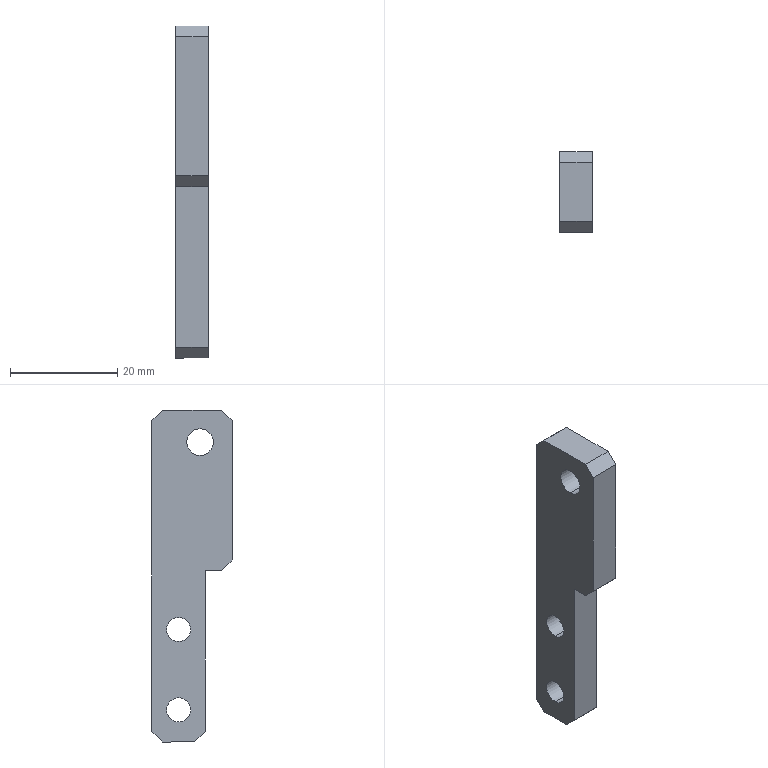Component | SolidWorks | 312981193FloatingJointConnection-1 | 1 solid | 19 faces | box 6 x 15 x 62 mm | volume 4251 mm3 | plane 13 | cylinder 6 | commonest cylinder face diameters 4.5 x4 5 x2 | material Q235-A
build123d program:
from build123d import *

# Parameters (mm, degrees)
BOSS_EXTRUDE1_DEPTH  = 6
M5_TAPPED_HOLE1_D    = 5
CHAMFER1_SIZE        = 2
M4_CLEARANCE_HOLE1_D = 4.5


with BuildPart() as part:
    # Sketch2 → Boss-Extrude1 (new body)
    with BuildSketch(Plane.XY):
        Polygon((-30, 15), (0, 15), (0, 0), (-62, 0), (-62, 10), (-30, 10), align=None)
    extrude(amount=BOSS_EXTRUDE1_DEPTH)

    # M5 Tapped Hole1 (through all)
    with Locations(Plane.XY.offset(6)):
        with Locations((-6, 9)):
            Hole(M5_TAPPED_HOLE1_D / 2)

    # Chamfer1
    chamfer1_edges = [part.edges().sort_by_distance(p)[0] for p in [
        (-30, 15, 3),
        (0, 15, 3),
        (0, 0, 3),
        (-62, 0, 3),
        (-62, 10, 3),
    ]]
    chamfer(chamfer1_edges, length=CHAMFER1_SIZE)

    # M4 Clearance Hole1 (through all)
    with Locations(Plane.XY.offset(6)):
        with Locations((-56, 5), (-41, 5)):
            Hole(M4_CLEARANCE_HOLE1_D / 2)


solid = part.part

# Placed as in the assembly
solid = solid.moved(Location((143.77, 31.768, 86.829), (180, 90, 0)))
STEP:
#1=CARTESIAN_POINT('',(5.66,1.054,1.125));
#2=VERTEX_POINT('',#1);
#3=CARTESIAN_POINT('',(5.66,1.054,1.302));
#4=VERTEX_POINT('',#3);
#5=CARTESIAN_POINT('',(5.66,1.054,1.214));
#6=DIRECTION('',(1.,0.,0.));
#7=DIRECTION('',(0.,0.,1.));
#8=AXIS2_PLACEMENT_3D('',#5,#6,#7);
#9=CIRCLE('',#8,0.08858);
#10=EDGE_CURVE('',#2,#4,#9,.T.);
#11=ORIENTED_EDGE('',*,*,#10,.F.);
#12=CARTESIAN_POINT('',(5.896,1.054,1.125));
#13=VERTEX_POINT('',#12);
#14=CARTESIAN_POINT('',(5.896,1.054,1.125));
#15=DIRECTION('',(1.,0.,0.));
#16=VECTOR('',#15,39.37);
#17=LINE('',#14,#16);
#18=EDGE_CURVE('',#2,#13,#17,.T.);
#19=ORIENTED_EDGE('',*,*,#18,.T.);
#20=CARTESIAN_POINT('',(5.896,1.054,1.302));
#21=VERTEX_POINT('',#20);
#22=CARTESIAN_POINT('',(5.896,1.054,1.214));
#23=DIRECTION('',(1.,0.,0.));
#24=DIRECTION('',(0.,0.,1.));
#25=AXIS2_PLACEMENT_3D('',#22,#23,#24);
#26=CIRCLE('',#25,0.08858);
#27=EDGE_CURVE('',#13,#21,#26,.T.);
#28=ORIENTED_EDGE('',*,*,#27,.T.);
#29=CARTESIAN_POINT('',(5.896,1.054,1.302));
#30=DIRECTION('',(1.,0.,0.));
#31=VECTOR('',#30,39.37);
#32=LINE('',#29,#31);
#33=EDGE_CURVE('',#4,#21,#32,.T.);
#34=ORIENTED_EDGE('',*,*,#33,.F.);
#35=EDGE_LOOP('',(#11,#19,#28,#34));
#36=FACE_OUTER_BOUND('',#35,.T.);
#37=CARTESIAN_POINT('',(5.896,1.054,1.214));
#38=DIRECTION('',(1.,0.,0.));
#39=DIRECTION('',(0.,0.,1.));
#40=AXIS2_PLACEMENT_3D('',#37,#38,#39);
#41=CYLINDRICAL_SURFACE('',#40,0.08858);
#42=ADVANCED_FACE('',(#36),#41,.F.);
#43=CARTESIAN_POINT('',(5.66,1.054,1.716));
#44=VERTEX_POINT('',#43);
#45=CARTESIAN_POINT('',(5.66,1.054,1.893));
#46=VERTEX_POINT('',#45);
#47=CARTESIAN_POINT('',(5.66,1.054,1.804));
#48=DIRECTION('',(1.,0.,0.));
#49=DIRECTION('',(0.,0.,1.));
#50=AXIS2_PLACEMENT_3D('',#47,#48,#49);
#51=CIRCLE('',#50,0.08858);
#52=EDGE_CURVE('',#44,#46,#51,.T.);
#53=ORIENTED_EDGE('',*,*,#52,.F.);
#54=CARTESIAN_POINT('',(5.896,1.054,1.716));
#55=VERTEX_POINT('',#54);
#56=CARTESIAN_POINT('',(5.896,1.054,1.716));
#57=DIRECTION('',(1.,0.,0.));
#58=VECTOR('',#57,39.37);
#59=LINE('',#56,#58);
#60=EDGE_CURVE('',#44,#55,#59,.T.);
#61=ORIENTED_EDGE('',*,*,#60,.T.);
#62=CARTESIAN_POINT('',(5.896,1.054,1.893));
#63=VERTEX_POINT('',#62);
#64=CARTESIAN_POINT('',(5.896,1.054,1.804));
#65=DIRECTION('',(1.,0.,0.));
#66=DIRECTION('',(0.,0.,1.));
#67=AXIS2_PLACEMENT_3D('',#64,#65,#66);
#68=CIRCLE('',#67,0.08858);
#69=EDGE_CURVE('',#55,#63,#68,.T.);
#70=ORIENTED_EDGE('',*,*,#69,.T.);
#71=CARTESIAN_POINT('',(5.896,1.054,1.893));
#72=DIRECTION('',(1.,0.,0.));
#73=VECTOR('',#72,39.37);
#74=LINE('',#71,#73);
#75=EDGE_CURVE('',#46,#63,#74,.T.);
#76=ORIENTED_EDGE('',*,*,#75,.F.);
#77=EDGE_LOOP('',(#53,#61,#70,#76));
#78=FACE_OUTER_BOUND('',#77,.T.);
#79=CARTESIAN_POINT('',(5.896,1.054,1.804));
#80=DIRECTION('',(1.,0.,0.));
#81=DIRECTION('',(0.,0.,1.));
#82=AXIS2_PLACEMENT_3D('',#79,#80,#81);
#83=CYLINDRICAL_SURFACE('',#82,0.08858);
#84=ADVANCED_FACE('',(#78),#83,.F.);
#85=CARTESIAN_POINT('',(5.66,0.8964,3.084));
#86=VERTEX_POINT('',#85);
#87=CARTESIAN_POINT('',(5.66,0.8964,3.281));
#88=VERTEX_POINT('',#87);
#89=CARTESIAN_POINT('',(5.66,0.8964,3.182));
#90=DIRECTION('',(1.,0.,0.));
#91=DIRECTION('',(0.,0.,1.));
#92=AXIS2_PLACEMENT_3D('',#89,#90,#91);
#93=CIRCLE('',#92,0.09843);
#94=EDGE_CURVE('',#86,#88,#93,.T.);
#95=ORIENTED_EDGE('',*,*,#94,.F.);
#96=CARTESIAN_POINT('',(5.896,0.8964,3.084));
#97=VERTEX_POINT('',#96);
#98=CARTESIAN_POINT('',(5.896,0.8964,3.084));
#99=DIRECTION('',(1.,0.,0.));
#100=VECTOR('',#99,39.37);
#101=LINE('',#98,#100);
#102=EDGE_CURVE('',#86,#97,#101,.T.);
#103=ORIENTED_EDGE('',*,*,#102,.T.);
#104=CARTESIAN_POINT('',(5.896,0.8964,3.281));
#105=VERTEX_POINT('',#104);
#106=CARTESIAN_POINT('',(5.896,0.8964,3.182));
#107=DIRECTION('',(1.,0.,0.));
#108=DIRECTION('',(0.,0.,1.));
#109=AXIS2_PLACEMENT_3D('',#106,#107,#108);
#110=CIRCLE('',#109,0.09843);
#111=EDGE_CURVE('',#97,#105,#110,.T.);
#112=ORIENTED_EDGE('',*,*,#111,.T.);
#113=CARTESIAN_POINT('',(5.896,0.8964,3.281));
#114=DIRECTION('',(1.,0.,0.));
#115=VECTOR('',#114,39.37);
#116=LINE('',#113,#115);
#117=EDGE_CURVE('',#88,#105,#116,.T.);
#118=ORIENTED_EDGE('',*,*,#117,.F.);
#119=EDGE_LOOP('',(#95,#103,#112,#118));
#120=FACE_OUTER_BOUND('',#119,.T.);
#121=CARTESIAN_POINT('',(5.896,0.8964,3.182));
#122=DIRECTION('',(1.,0.,0.));
#123=DIRECTION('',(0.,0.,1.));
#124=AXIS2_PLACEMENT_3D('',#121,#122,#123);
#125=CYLINDRICAL_SURFACE('',#124,0.09843);
#126=ADVANCED_FACE('',(#120),#125,.F.);
#127=CARTESIAN_POINT('',(5.896,0.7389,2.237));
#128=VERTEX_POINT('',#127);
#129=CARTESIAN_POINT('',(5.896,0.857,2.237));
#130=VERTEX_POINT('',#129);
#131=CARTESIAN_POINT('',(5.896,0.6602,2.237));
#132=DIRECTION('',(-0.,1.,-0.));
#133=VECTOR('',#132,39.37);
#134=LINE('',#131,#133);
#135=EDGE_CURVE('',#128,#130,#134,.T.);
#136=ORIENTED_EDGE('',*,*,#135,.F.);
#137=CARTESIAN_POINT('',(5.66,0.7389,2.237));
#138=VERTEX_POINT('',#137);
#139=CARTESIAN_POINT('',(5.896,0.7389,2.237));
#140=DIRECTION('',(-1.,-0.,-0.));
#141=VECTOR('',#140,39.37);
#142=LINE('',#139,#141);
#143=EDGE_CURVE('',#128,#138,#142,.T.);
#144=ORIENTED_EDGE('',*,*,#143,.T.);
#145=CARTESIAN_POINT('',(5.66,0.857,2.237));
#146=VERTEX_POINT('',#145);
#147=CARTESIAN_POINT('',(5.66,0.6602,2.237));
#148=DIRECTION('',(-0.,1.,-0.));
#149=VECTOR('',#148,39.37);
#150=LINE('',#147,#149);
#151=EDGE_CURVE('',#138,#146,#150,.T.);
#152=ORIENTED_EDGE('',*,*,#151,.T.);
#153=CARTESIAN_POINT('',(5.896,0.857,2.237));
#154=DIRECTION('',(-1.,-0.,-0.));
#155=VECTOR('',#154,39.37);
#156=LINE('',#153,#155);
#157=EDGE_CURVE('',#130,#146,#156,.T.);
#158=ORIENTED_EDGE('',*,*,#157,.F.);
#159=EDGE_LOOP('',(#136,#144,#152,#158));
#160=FACE_OUTER_BOUND('',#159,.T.);
#161=CARTESIAN_POINT('',(5.896,0.6602,2.237));
#162=DIRECTION('',(-0.,0.,1.));
#163=DIRECTION('',(-1.,-0.,-0.));
#164=AXIS2_PLACEMENT_3D('',#161,#162,#163);
#165=PLANE('',#164);
#166=ADVANCED_FACE('',(#160),#165,.F.);
#167=CARTESIAN_POINT('',(5.66,0.857,1.056));
#168=VERTEX_POINT('',#167);
#169=CARTESIAN_POINT('',(5.66,0.857,0.9775));
#170=DIRECTION('',(0.,-0.,-1.));
#171=VECTOR('',#170,39.37);
#172=LINE('',#169,#171);
#173=EDGE_CURVE('',#146,#168,#172,.T.);
#174=ORIENTED_EDGE('',*,*,#173,.T.);
#175=CARTESIAN_POINT('',(5.896,0.857,1.056));
#176=VERTEX_POINT('',#175);
#177=CARTESIAN_POINT('',(5.896,0.857,1.056));
#178=DIRECTION('',(1.,0.,0.));
#179=VECTOR('',#178,39.37);
#180=LINE('',#177,#179);
#181=EDGE_CURVE('',#168,#176,#180,.T.);
#182=ORIENTED_EDGE('',*,*,#181,.T.);
#183=CARTESIAN_POINT('',(5.896,0.857,0.9775));
#184=DIRECTION('',(0.,-0.,-1.));
#185=VECTOR('',#184,39.37);
#186=LINE('',#183,#185);
#187=EDGE_CURVE('',#130,#176,#186,.T.);
#188=ORIENTED_EDGE('',*,*,#187,.F.);
#189=ORIENTED_EDGE('',*,*,#157,.T.);
#190=EDGE_LOOP('',(#174,#182,#188,#189));
#191=FACE_OUTER_BOUND('',#190,.T.);
#192=CARTESIAN_POINT('',(5.896,0.857,0.9775));
#193=DIRECTION('',(-0.,1.,-0.));
#194=DIRECTION('',(-1.,-0.,-0.));
#195=AXIS2_PLACEMENT_3D('',#192,#193,#194);
#196=PLANE('',#195);
#197=ADVANCED_FACE('',(#191),#196,.F.);
#198=CARTESIAN_POINT('',(5.66,0.9358,0.9775));
#199=VERTEX_POINT('',#198);
#200=CARTESIAN_POINT('',(5.66,1.172,0.9775));
#201=VERTEX_POINT('',#200);
#202=CARTESIAN_POINT('',(5.66,1.251,0.9775));
#203=DIRECTION('',(-0.,1.,-0.));
#204=VECTOR('',#203,39.37);
#205=LINE('',#202,#204);
#206=EDGE_CURVE('',#199,#201,#205,.T.);
#207=ORIENTED_EDGE('',*,*,#206,.T.);
#208=CARTESIAN_POINT('',(5.896,1.172,0.9775));
#209=VERTEX_POINT('',#208);
#210=CARTESIAN_POINT('',(5.896,1.172,0.9775));
#211=DIRECTION('',(1.,0.,0.));
#212=VECTOR('',#211,39.37);
#213=LINE('',#210,#212);
#214=EDGE_CURVE('',#201,#209,#213,.T.);
#215=ORIENTED_EDGE('',*,*,#214,.T.);
#216=CARTESIAN_POINT('',(5.896,0.9358,0.9775));
#217=VERTEX_POINT('',#216);
#218=CARTESIAN_POINT('',(5.896,1.251,0.9775));
#219=DIRECTION('',(-0.,1.,-0.));
#220=VECTOR('',#219,39.37);
#221=LINE('',#218,#220);
#222=EDGE_CURVE('',#217,#209,#221,.T.);
#223=ORIENTED_EDGE('',*,*,#222,.F.);
#224=CARTESIAN_POINT('',(5.896,0.9358,0.9775));
#225=DIRECTION('',(-1.,-0.,-0.));
#226=VECTOR('',#225,39.37);
#227=LINE('',#224,#226);
#228=EDGE_CURVE('',#217,#199,#227,.T.);
#229=ORIENTED_EDGE('',*,*,#228,.T.);
#230=EDGE_LOOP('',(#207,#215,#223,#229));
#231=FACE_OUTER_BOUND('',#230,.T.);
#232=CARTESIAN_POINT('',(5.896,1.251,0.9775));
#233=DIRECTION('',(-0.,0.,1.));
#234=DIRECTION('',(-1.,-0.,-0.));
#235=AXIS2_PLACEMENT_3D('',#232,#233,#234);
#236=PLANE('',#235);
#237=ADVANCED_FACE('',(#231),#236,.F.);
#238=CARTESIAN_POINT('',(5.896,1.251,1.056));
#239=VERTEX_POINT('',#238);
#240=CARTESIAN_POINT('',(5.896,1.251,3.34));
#241=VERTEX_POINT('',#240);
#242=CARTESIAN_POINT('',(5.896,1.251,0.9775));
#243=DIRECTION('',(-0.,0.,1.));
#244=VECTOR('',#243,39.37);
#245=LINE('',#242,#244);
#246=EDGE_CURVE('',#239,#241,#245,.T.);
#247=ORIENTED_EDGE('',*,*,#246,.F.);
#248=CARTESIAN_POINT('',(5.66,1.251,1.056));
#249=VERTEX_POINT('',#248);
#250=CARTESIAN_POINT('',(5.896,1.251,1.056));
#251=DIRECTION('',(-1.,-0.,-0.));
#252=VECTOR('',#251,39.37);
#253=LINE('',#250,#252);
#254=EDGE_CURVE('',#239,#249,#253,.T.);
#255=ORIENTED_EDGE('',*,*,#254,.T.);
#256=CARTESIAN_POINT('',(5.66,1.251,3.34));
#257=VERTEX_POINT('',#256);
#258=CARTESIAN_POINT('',(5.66,1.251,0.9775));
#259=DIRECTION('',(-0.,0.,1.));
#260=VECTOR('',#259,39.37);
#261=LINE('',#258,#260);
#262=EDGE_CURVE('',#249,#257,#261,.T.);
#263=ORIENTED_EDGE('',*,*,#262,.T.);
#264=CARTESIAN_POINT('',(5.896,1.251,3.34));
#265=DIRECTION('',(1.,0.,0.));
#266=VECTOR('',#265,39.37);
#267=LINE('',#264,#266);
#268=EDGE_CURVE('',#257,#241,#267,.T.);
#269=ORIENTED_EDGE('',*,*,#268,.T.);
#270=EDGE_LOOP('',(#247,#255,#263,#269));
#271=FACE_OUTER_BOUND('',#270,.T.);
#272=CARTESIAN_POINT('',(5.896,1.251,0.9775));
#273=DIRECTION('',(0.,-1.,0.));
#274=DIRECTION('',(1.,0.,0.));
#275=AXIS2_PLACEMENT_3D('',#272,#273,#274);
#276=PLANE('',#275);
#277=ADVANCED_FACE('',(#271),#276,.F.);
#278=CARTESIAN_POINT('',(5.896,1.172,3.418));
#279=VERTEX_POINT('',#278);
#280=CARTESIAN_POINT('',(5.896,0.7389,3.418));
#281=VERTEX_POINT('',#280);
#282=CARTESIAN_POINT('',(5.896,0.6602,3.418));
#283=DIRECTION('',(0.,-1.,0.));
#284=VECTOR('',#283,39.37);
#285=LINE('',#282,#284);
#286=EDGE_CURVE('',#279,#281,#285,.T.);
#287=ORIENTED_EDGE('',*,*,#286,.F.);
#288=CARTESIAN_POINT('',(5.66,1.172,3.418));
#289=VERTEX_POINT('',#288);
#290=CARTESIAN_POINT('',(5.896,1.172,3.418));
#291=DIRECTION('',(-1.,-0.,-0.));
#292=VECTOR('',#291,39.37);
#293=LINE('',#290,#292);
#294=EDGE_CURVE('',#279,#289,#293,.T.);
#295=ORIENTED_EDGE('',*,*,#294,.T.);
#296=CARTESIAN_POINT('',(5.66,0.7389,3.418));
#297=VERTEX_POINT('',#296);
#298=CARTESIAN_POINT('',(5.66,0.6602,3.418));
#299=DIRECTION('',(0.,-1.,0.));
#300=VECTOR('',#299,39.37);
#301=LINE('',#298,#300);
#302=EDGE_CURVE('',#289,#297,#301,.T.);
#303=ORIENTED_EDGE('',*,*,#302,.T.);
#304=CARTESIAN_POINT('',(5.896,0.7389,3.418));
#305=DIRECTION('',(1.,0.,0.));
#306=VECTOR('',#305,39.37);
#307=LINE('',#304,#306);
#308=EDGE_CURVE('',#297,#281,#307,.T.);
#309=ORIENTED_EDGE('',*,*,#308,.T.);
#310=EDGE_LOOP('',(#287,#295,#303,#309));
#311=FACE_OUTER_BOUND('',#310,.T.);
#312=CARTESIAN_POINT('',(5.896,0.6602,3.418));
#313=DIRECTION('',(0.,-0.,-1.));
#314=DIRECTION('',(-0.,1.,-0.));
#315=AXIS2_PLACEMENT_3D('',#312,#313,#314);
#316=PLANE('',#315);
#317=ADVANCED_FACE('',(#311),#316,.F.);
#318=CARTESIAN_POINT('',(5.66,0.6602,3.34));
#319=VERTEX_POINT('',#318);
#320=CARTESIAN_POINT('',(5.66,0.6602,2.316));
#321=VERTEX_POINT('',#320);
#322=CARTESIAN_POINT('',(5.66,0.6602,2.237));
#323=DIRECTION('',(0.,-0.,-1.));
#324=VECTOR('',#323,39.37);
#325=LINE('',#322,#324);
#326=EDGE_CURVE('',#319,#321,#325,.T.);
#327=ORIENTED_EDGE('',*,*,#326,.T.);
#328=CARTESIAN_POINT('',(5.896,0.6602,2.316));
#329=VERTEX_POINT('',#328);
#330=CARTESIAN_POINT('',(5.896,0.6602,2.316));
#331=DIRECTION('',(1.,0.,0.));
#332=VECTOR('',#331,39.37);
#333=LINE('',#330,#332);
#334=EDGE_CURVE('',#321,#329,#333,.T.);
#335=ORIENTED_EDGE('',*,*,#334,.T.);
#336=CARTESIAN_POINT('',(5.896,0.6602,3.34));
#337=VERTEX_POINT('',#336);
#338=CARTESIAN_POINT('',(5.896,0.6602,2.237));
#339=DIRECTION('',(0.,-0.,-1.));
#340=VECTOR('',#339,39.37);
#341=LINE('',#338,#340);
#342=EDGE_CURVE('',#337,#329,#341,.T.);
#343=ORIENTED_EDGE('',*,*,#342,.F.);
#344=CARTESIAN_POINT('',(5.896,0.6602,3.34));
#345=DIRECTION('',(-1.,-0.,-0.));
#346=VECTOR('',#345,39.37);
#347=LINE('',#344,#346);
#348=EDGE_CURVE('',#337,#319,#347,.T.);
#349=ORIENTED_EDGE('',*,*,#348,.T.);
#350=EDGE_LOOP('',(#327,#335,#343,#349));
#351=FACE_OUTER_BOUND('',#350,.T.);
#352=CARTESIAN_POINT('',(5.896,0.6602,2.237));
#353=DIRECTION('',(-0.,1.,-0.));
#354=DIRECTION('',(-1.,-0.,-0.));
#355=AXIS2_PLACEMENT_3D('',#352,#353,#354);
#356=PLANE('',#355);
#357=ADVANCED_FACE('',(#351),#356,.F.);
#358=CARTESIAN_POINT('',(5.896,1.054,1.214));
#359=DIRECTION('',(1.,0.,0.));
#360=DIRECTION('',(0.,0.,1.));
#361=AXIS2_PLACEMENT_3D('',#358,#359,#360);
#362=CIRCLE('',#361,0.08858);
#363=EDGE_CURVE('',#21,#13,#362,.T.);
#364=ORIENTED_EDGE('',*,*,#363,.F.);
#365=ORIENTED_EDGE('',*,*,#27,.F.);
#366=EDGE_LOOP('',(#364,#365));
#367=FACE_BOUND('',#366,.T.);
#368=CARTESIAN_POINT('',(5.896,1.054,1.804));
#369=DIRECTION('',(1.,0.,0.));
#370=DIRECTION('',(0.,0.,1.));
#371=AXIS2_PLACEMENT_3D('',#368,#369,#370);
#372=CIRCLE('',#371,0.08858);
#373=EDGE_CURVE('',#63,#55,#372,.T.);
#374=ORIENTED_EDGE('',*,*,#373,.F.);
#375=ORIENTED_EDGE('',*,*,#69,.F.);
#376=EDGE_LOOP('',(#374,#375));
#377=FACE_BOUND('',#376,.T.);
#378=CARTESIAN_POINT('',(5.896,0.8964,3.182));
#379=DIRECTION('',(1.,0.,0.));
#380=DIRECTION('',(0.,0.,1.));
#381=AXIS2_PLACEMENT_3D('',#378,#379,#380);
#382=CIRCLE('',#381,0.09843);
#383=EDGE_CURVE('',#105,#97,#382,.T.);
#384=ORIENTED_EDGE('',*,*,#383,.F.);
#385=ORIENTED_EDGE('',*,*,#111,.F.);
#386=EDGE_LOOP('',(#384,#385));
#387=FACE_BOUND('',#386,.T.);
#388=ORIENTED_EDGE('',*,*,#222,.T.);
#389=CARTESIAN_POINT('',(5.896,1.644,1.45));
#390=DIRECTION('',(-0.,0.7071,0.7071));
#391=VECTOR('',#390,39.37);
#392=LINE('',#389,#391);
#393=EDGE_CURVE('',#209,#239,#392,.T.);
#394=ORIENTED_EDGE('',*,*,#393,.T.);
#395=ORIENTED_EDGE('',*,*,#246,.T.);
#396=CARTESIAN_POINT('',(5.896,1.605,2.985));
#397=DIRECTION('',(-0.,-0.7071,0.7071));
#398=VECTOR('',#397,39.37);
#399=LINE('',#396,#398);
#400=EDGE_CURVE('',#241,#279,#399,.T.);
#401=ORIENTED_EDGE('',*,*,#400,.T.);
#402=ORIENTED_EDGE('',*,*,#286,.T.);
#403=CARTESIAN_POINT('',(5.896,0.2074,2.887));
#404=DIRECTION('',(0.,-0.7071,-0.7071));
#405=VECTOR('',#404,39.37);
#406=LINE('',#403,#405);
#407=EDGE_CURVE('',#281,#337,#406,.T.);
#408=ORIENTED_EDGE('',*,*,#407,.T.);
#409=ORIENTED_EDGE('',*,*,#342,.T.);
#410=CARTESIAN_POINT('',(5.896,0.798,2.178));
#411=DIRECTION('',(0.,0.7071,-0.7071));
#412=VECTOR('',#411,39.37);
#413=LINE('',#410,#412);
#414=EDGE_CURVE('',#329,#128,#413,.T.);
#415=ORIENTED_EDGE('',*,*,#414,.T.);
#416=ORIENTED_EDGE('',*,*,#135,.T.);
#417=ORIENTED_EDGE('',*,*,#187,.T.);
#418=CARTESIAN_POINT('',(5.896,0.2665,1.647));
#419=DIRECTION('',(0.,0.7071,-0.7071));
#420=VECTOR('',#419,39.37);
#421=LINE('',#418,#420);
#422=EDGE_CURVE('',#176,#217,#421,.T.);
#423=ORIENTED_EDGE('',*,*,#422,.T.);
#424=EDGE_LOOP('',(#388,#394,#395,#401,#402,#408,#409,#415,#416,#417,#423));
#425=FACE_OUTER_BOUND('',#424,.T.);
#426=CARTESIAN_POINT('',(5.896,0.857,2.237));
#427=DIRECTION('',(1.,0.,0.));
#428=DIRECTION('',(-0.,0.,1.));
#429=AXIS2_PLACEMENT_3D('',#426,#427,#428);
#430=PLANE('',#429);
#431=ADVANCED_FACE('',(#367,#377,#387,#425),#430,.T.);
#432=CARTESIAN_POINT('',(5.66,1.054,1.214));
#433=DIRECTION('',(1.,0.,0.));
#434=DIRECTION('',(0.,0.,1.));
#435=AXIS2_PLACEMENT_3D('',#432,#433,#434);
#436=CIRCLE('',#435,0.08858);
#437=EDGE_CURVE('',#4,#2,#436,.T.);
#438=ORIENTED_EDGE('',*,*,#437,.T.);
#439=ORIENTED_EDGE('',*,*,#10,.T.);
#440=EDGE_LOOP('',(#438,#439));
#441=FACE_BOUND('',#440,.T.);
#442=CARTESIAN_POINT('',(5.66,1.054,1.804));
#443=DIRECTION('',(1.,0.,0.));
#444=DIRECTION('',(0.,0.,1.));
#445=AXIS2_PLACEMENT_3D('',#442,#443,#444);
#446=CIRCLE('',#445,0.08858);
#447=EDGE_CURVE('',#46,#44,#446,.T.);
#448=ORIENTED_EDGE('',*,*,#447,.T.);
#449=ORIENTED_EDGE('',*,*,#52,.T.);
#450=EDGE_LOOP('',(#448,#449));
#451=FACE_BOUND('',#450,.T.);
#452=CARTESIAN_POINT('',(5.66,0.8964,3.182));
#453=DIRECTION('',(1.,0.,0.));
#454=DIRECTION('',(0.,0.,1.));
#455=AXIS2_PLACEMENT_3D('',#452,#453,#454);
#456=CIRCLE('',#455,0.09843);
#457=EDGE_CURVE('',#88,#86,#456,.T.);
#458=ORIENTED_EDGE('',*,*,#457,.T.);
#459=ORIENTED_EDGE('',*,*,#94,.T.);
#460=EDGE_LOOP('',(#458,#459));
#461=FACE_BOUND('',#460,.T.);
#462=ORIENTED_EDGE('',*,*,#262,.F.);
#463=CARTESIAN_POINT('',(5.66,1.251,1.056));
#464=DIRECTION('',(0.,-0.7071,-0.7071));
#465=VECTOR('',#464,39.37);
#466=LINE('',#463,#465);
#467=EDGE_CURVE('',#249,#201,#466,.T.);
#468=ORIENTED_EDGE('',*,*,#467,.T.);
#469=ORIENTED_EDGE('',*,*,#206,.F.);
#470=CARTESIAN_POINT('',(5.66,0.9358,0.9775));
#471=DIRECTION('',(-0.,-0.7071,0.7071));
#472=VECTOR('',#471,39.37);
#473=LINE('',#470,#472);
#474=EDGE_CURVE('',#199,#168,#473,.T.);
#475=ORIENTED_EDGE('',*,*,#474,.T.);
#476=ORIENTED_EDGE('',*,*,#173,.F.);
#477=ORIENTED_EDGE('',*,*,#151,.F.);
#478=CARTESIAN_POINT('',(5.66,0.7389,2.237));
#479=DIRECTION('',(-0.,-0.7071,0.7071));
#480=VECTOR('',#479,39.37);
#481=LINE('',#478,#480);
#482=EDGE_CURVE('',#138,#321,#481,.T.);
#483=ORIENTED_EDGE('',*,*,#482,.T.);
#484=ORIENTED_EDGE('',*,*,#326,.F.);
#485=CARTESIAN_POINT('',(5.66,0.6602,3.34));
#486=DIRECTION('',(-0.,0.7071,0.7071));
#487=VECTOR('',#486,39.37);
#488=LINE('',#485,#487);
#489=EDGE_CURVE('',#319,#297,#488,.T.);
#490=ORIENTED_EDGE('',*,*,#489,.T.);
#491=ORIENTED_EDGE('',*,*,#302,.F.);
#492=CARTESIAN_POINT('',(5.66,1.172,3.418));
#493=DIRECTION('',(0.,0.7071,-0.7071));
#494=VECTOR('',#493,39.37);
#495=LINE('',#492,#494);
#496=EDGE_CURVE('',#289,#257,#495,.T.);
#497=ORIENTED_EDGE('',*,*,#496,.T.);
#498=EDGE_LOOP('',(#462,#468,#469,#475,#476,#477,#483,#484,#490,#491,#497));
#499=FACE_OUTER_BOUND('',#498,.T.);
#500=CARTESIAN_POINT('',(5.66,0.857,2.237));
#501=DIRECTION('',(1.,0.,0.));
#502=DIRECTION('',(-0.,0.,1.));
#503=AXIS2_PLACEMENT_3D('',#500,#501,#502);
#504=PLANE('',#503);
#505=ADVANCED_FACE('',(#441,#451,#461,#499),#504,.F.);
#506=ORIENTED_EDGE('',*,*,#102,.F.);
#507=ORIENTED_EDGE('',*,*,#457,.F.);
#508=ORIENTED_EDGE('',*,*,#117,.T.);
#509=ORIENTED_EDGE('',*,*,#383,.T.);
#510=EDGE_LOOP('',(#506,#507,#508,#509));
#511=FACE_OUTER_BOUND('',#510,.T.);
#512=CARTESIAN_POINT('',(5.896,0.8964,3.182));
#513=DIRECTION('',(1.,0.,0.));
#514=DIRECTION('',(0.,0.,1.));
#515=AXIS2_PLACEMENT_3D('',#512,#513,#514);
#516=CYLINDRICAL_SURFACE('',#515,0.09843);
#517=ADVANCED_FACE('',(#511),#516,.F.);
#518=ORIENTED_EDGE('',*,*,#393,.F.);
#519=ORIENTED_EDGE('',*,*,#214,.F.);
#520=ORIENTED_EDGE('',*,*,#467,.F.);
#521=ORIENTED_EDGE('',*,*,#254,.F.);
#522=EDGE_LOOP('',(#518,#519,#520,#521));
#523=FACE_OUTER_BOUND('',#522,.T.);
#524=CARTESIAN_POINT('',(5.896,1.251,1.056));
#525=DIRECTION('',(-0.,-0.7071,0.7071));
#526=DIRECTION('',(0.,-0.7071,-0.7071));
#527=AXIS2_PLACEMENT_3D('',#524,#525,#526);
#528=PLANE('',#527);
#529=ADVANCED_FACE('',(#523),#528,.F.);
#530=ORIENTED_EDGE('',*,*,#422,.F.);
#531=ORIENTED_EDGE('',*,*,#181,.F.);
#532=ORIENTED_EDGE('',*,*,#474,.F.);
#533=ORIENTED_EDGE('',*,*,#228,.F.);
#534=EDGE_LOOP('',(#530,#531,#532,#533));
#535=FACE_OUTER_BOUND('',#534,.T.);
#536=CARTESIAN_POINT('',(5.896,0.9358,0.9775));
#537=DIRECTION('',(-0.,0.7071,0.7071));
#538=DIRECTION('',(-0.,-0.7071,0.7071));
#539=AXIS2_PLACEMENT_3D('',#536,#537,#538);
#540=PLANE('',#539);
#541=ADVANCED_FACE('',(#535),#540,.F.);
#542=ORIENTED_EDGE('',*,*,#414,.F.);
#543=ORIENTED_EDGE('',*,*,#334,.F.);
#544=ORIENTED_EDGE('',*,*,#482,.F.);
#545=ORIENTED_EDGE('',*,*,#143,.F.);
#546=EDGE_LOOP('',(#542,#543,#544,#545));
#547=FACE_OUTER_BOUND('',#546,.T.);
#548=CARTESIAN_POINT('',(5.896,0.7389,2.237));
#549=DIRECTION('',(-0.,0.7071,0.7071));
#550=DIRECTION('',(-0.,-0.7071,0.7071));
#551=AXIS2_PLACEMENT_3D('',#548,#549,#550);
#552=PLANE('',#551);
#553=ADVANCED_FACE('',(#547),#552,.F.);
#554=ORIENTED_EDGE('',*,*,#400,.F.);
#555=ORIENTED_EDGE('',*,*,#268,.F.);
#556=ORIENTED_EDGE('',*,*,#496,.F.);
#557=ORIENTED_EDGE('',*,*,#294,.F.);
#558=EDGE_LOOP('',(#554,#555,#556,#557));
#559=FACE_OUTER_BOUND('',#558,.T.);
#560=CARTESIAN_POINT('',(5.896,1.172,3.418));
#561=DIRECTION('',(0.,-0.7071,-0.7071));
#562=DIRECTION('',(0.,0.7071,-0.7071));
#563=AXIS2_PLACEMENT_3D('',#560,#561,#562);
#564=PLANE('',#563);
#565=ADVANCED_FACE('',(#559),#564,.F.);
#566=ORIENTED_EDGE('',*,*,#407,.F.);
#567=ORIENTED_EDGE('',*,*,#308,.F.);
#568=ORIENTED_EDGE('',*,*,#489,.F.);
#569=ORIENTED_EDGE('',*,*,#348,.F.);
#570=EDGE_LOOP('',(#566,#567,#568,#569));
#571=FACE_OUTER_BOUND('',#570,.T.);
#572=CARTESIAN_POINT('',(5.896,0.6602,3.34));
#573=DIRECTION('',(0.,0.7071,-0.7071));
#574=DIRECTION('',(-0.,0.7071,0.7071));
#575=AXIS2_PLACEMENT_3D('',#572,#573,#574);
#576=PLANE('',#575);
#577=ADVANCED_FACE('',(#571),#576,.F.);
#578=ORIENTED_EDGE('',*,*,#60,.F.);
#579=ORIENTED_EDGE('',*,*,#447,.F.);
#580=ORIENTED_EDGE('',*,*,#75,.T.);
#581=ORIENTED_EDGE('',*,*,#373,.T.);
#582=EDGE_LOOP('',(#578,#579,#580,#581));
#583=FACE_OUTER_BOUND('',#582,.T.);
#584=CARTESIAN_POINT('',(5.896,1.054,1.804));
#585=DIRECTION('',(1.,0.,0.));
#586=DIRECTION('',(0.,0.,1.));
#587=AXIS2_PLACEMENT_3D('',#584,#585,#586);
#588=CYLINDRICAL_SURFACE('',#587,0.08858);
#589=ADVANCED_FACE('',(#583),#588,.F.);
#590=ORIENTED_EDGE('',*,*,#18,.F.);
#591=ORIENTED_EDGE('',*,*,#437,.F.);
#592=ORIENTED_EDGE('',*,*,#33,.T.);
#593=ORIENTED_EDGE('',*,*,#363,.T.);
#594=EDGE_LOOP('',(#590,#591,#592,#593));
#595=FACE_OUTER_BOUND('',#594,.T.);
#596=CARTESIAN_POINT('',(5.896,1.054,1.214));
#597=DIRECTION('',(1.,0.,0.));
#598=DIRECTION('',(0.,0.,1.));
#599=AXIS2_PLACEMENT_3D('',#596,#597,#598);
#600=CYLINDRICAL_SURFACE('',#599,0.08858);
#601=ADVANCED_FACE('',(#595),#600,.F.);
#602=CLOSED_SHELL('',(#42,#84,#126,#166,#197,#237,#277,#317,#357,#431,#505,#517,#529,#541,#553,#565,#577,#589,#601));
#603=MANIFOLD_SOLID_BREP('',#602);
#604=CARTESIAN_POINT('',(0.,0.,0.));
#605=DIRECTION('',(0.,0.,1.));
#606=DIRECTION('',(1.,0.,0.));
#607=AXIS2_PLACEMENT_3D('',#604,#605,#606);
#608=(LENGTH_UNIT()NAMED_UNIT(*)SI_UNIT($,.METRE.));
#609=LENGTH_MEASURE_WITH_UNIT(LENGTH_MEASURE(0.0254),#608);
#610=DIMENSIONAL_EXPONENTS(1.,0.,0.,0.,0.,0.,0.);
#611=(CONVERSION_BASED_UNIT('',#609)LENGTH_UNIT()NAMED_UNIT(#610));
#612=UNCERTAINTY_MEASURE_WITH_UNIT(LENGTH_MEASURE(0.00001),#611,'','');
#613=(NAMED_UNIT(*)PLANE_ANGLE_UNIT()SI_UNIT($,.RADIAN.));
#614=(NAMED_UNIT(*)SI_UNIT($,.STERADIAN.)SOLID_ANGLE_UNIT());
#615=(GEOMETRIC_REPRESENTATION_CONTEXT(3)GLOBAL_UNCERTAINTY_ASSIGNED_CONTEXT((#612))GLOBAL_UNIT_ASSIGNED_CONTEXT((#611,#613,#614))REPRESENTATION_CONTEXT('',''));
#616=ADVANCED_BREP_SHAPE_REPRESENTATION('',(#603,#607),#615);
#617=COLOUR_RGB('',0.7922,0.8196,0.9333);
#618=FILL_AREA_STYLE_COLOUR('',#617);
#619=FILL_AREA_STYLE('',(#618));
#620=SURFACE_STYLE_FILL_AREA(#619);
#621=SURFACE_SIDE_STYLE('',(#620));
#622=SURFACE_STYLE_USAGE(.BOTH.,#621);
#623=PRESENTATION_STYLE_ASSIGNMENT((#622));
#624=STYLED_ITEM('',(#623),#603);
#625=PRESENTATION_LAYER_ASSIGNMENT('','',(#624));
#626=(LENGTH_UNIT()NAMED_UNIT(*)SI_UNIT($,.METRE.));
#627=LENGTH_MEASURE_WITH_UNIT(LENGTH_MEASURE(0.0254),#626);
#628=DIMENSIONAL_EXPONENTS(1.,0.,0.,0.,0.,0.,0.);
#629=(CONVERSION_BASED_UNIT('',#627)LENGTH_UNIT()NAMED_UNIT(#628));
#630=UNCERTAINTY_MEASURE_WITH_UNIT(LENGTH_MEASURE(0.00001),#629,'','');
#631=(NAMED_UNIT(*)PLANE_ANGLE_UNIT()SI_UNIT($,.RADIAN.));
#632=(NAMED_UNIT(*)SI_UNIT($,.STERADIAN.)SOLID_ANGLE_UNIT());
#633=(GEOMETRIC_REPRESENTATION_CONTEXT(3)GLOBAL_UNCERTAINTY_ASSIGNED_CONTEXT((#630))GLOBAL_UNIT_ASSIGNED_CONTEXT((#629,#631,#632))REPRESENTATION_CONTEXT('',''));
#634=MECHANICAL_DESIGN_GEOMETRIC_PRESENTATION_REPRESENTATION('',(#624),#633);